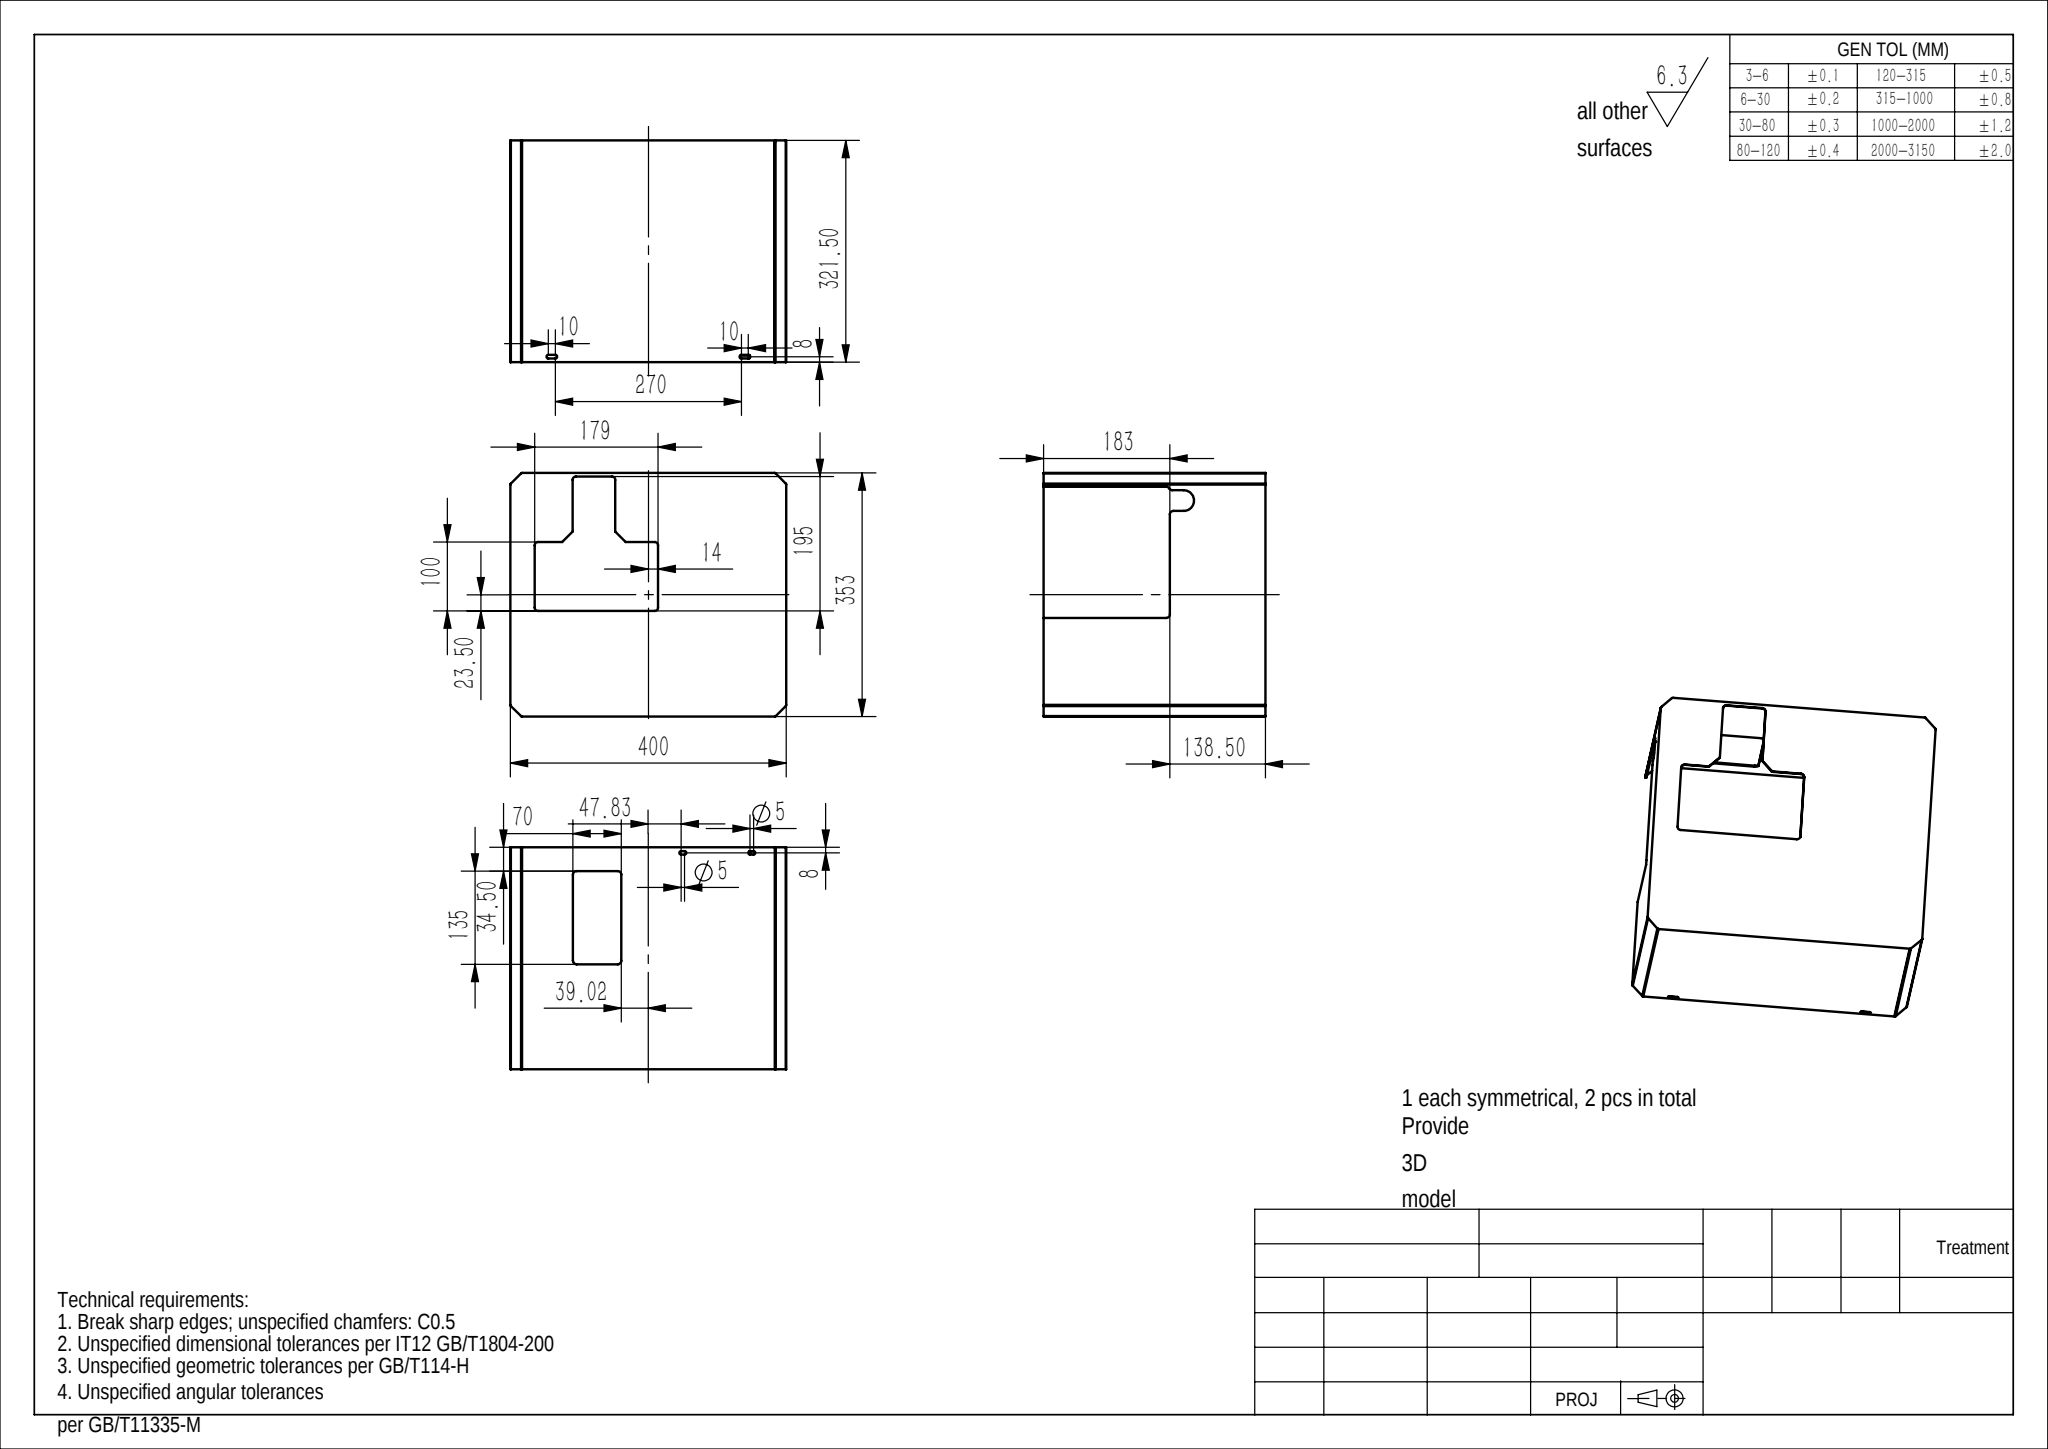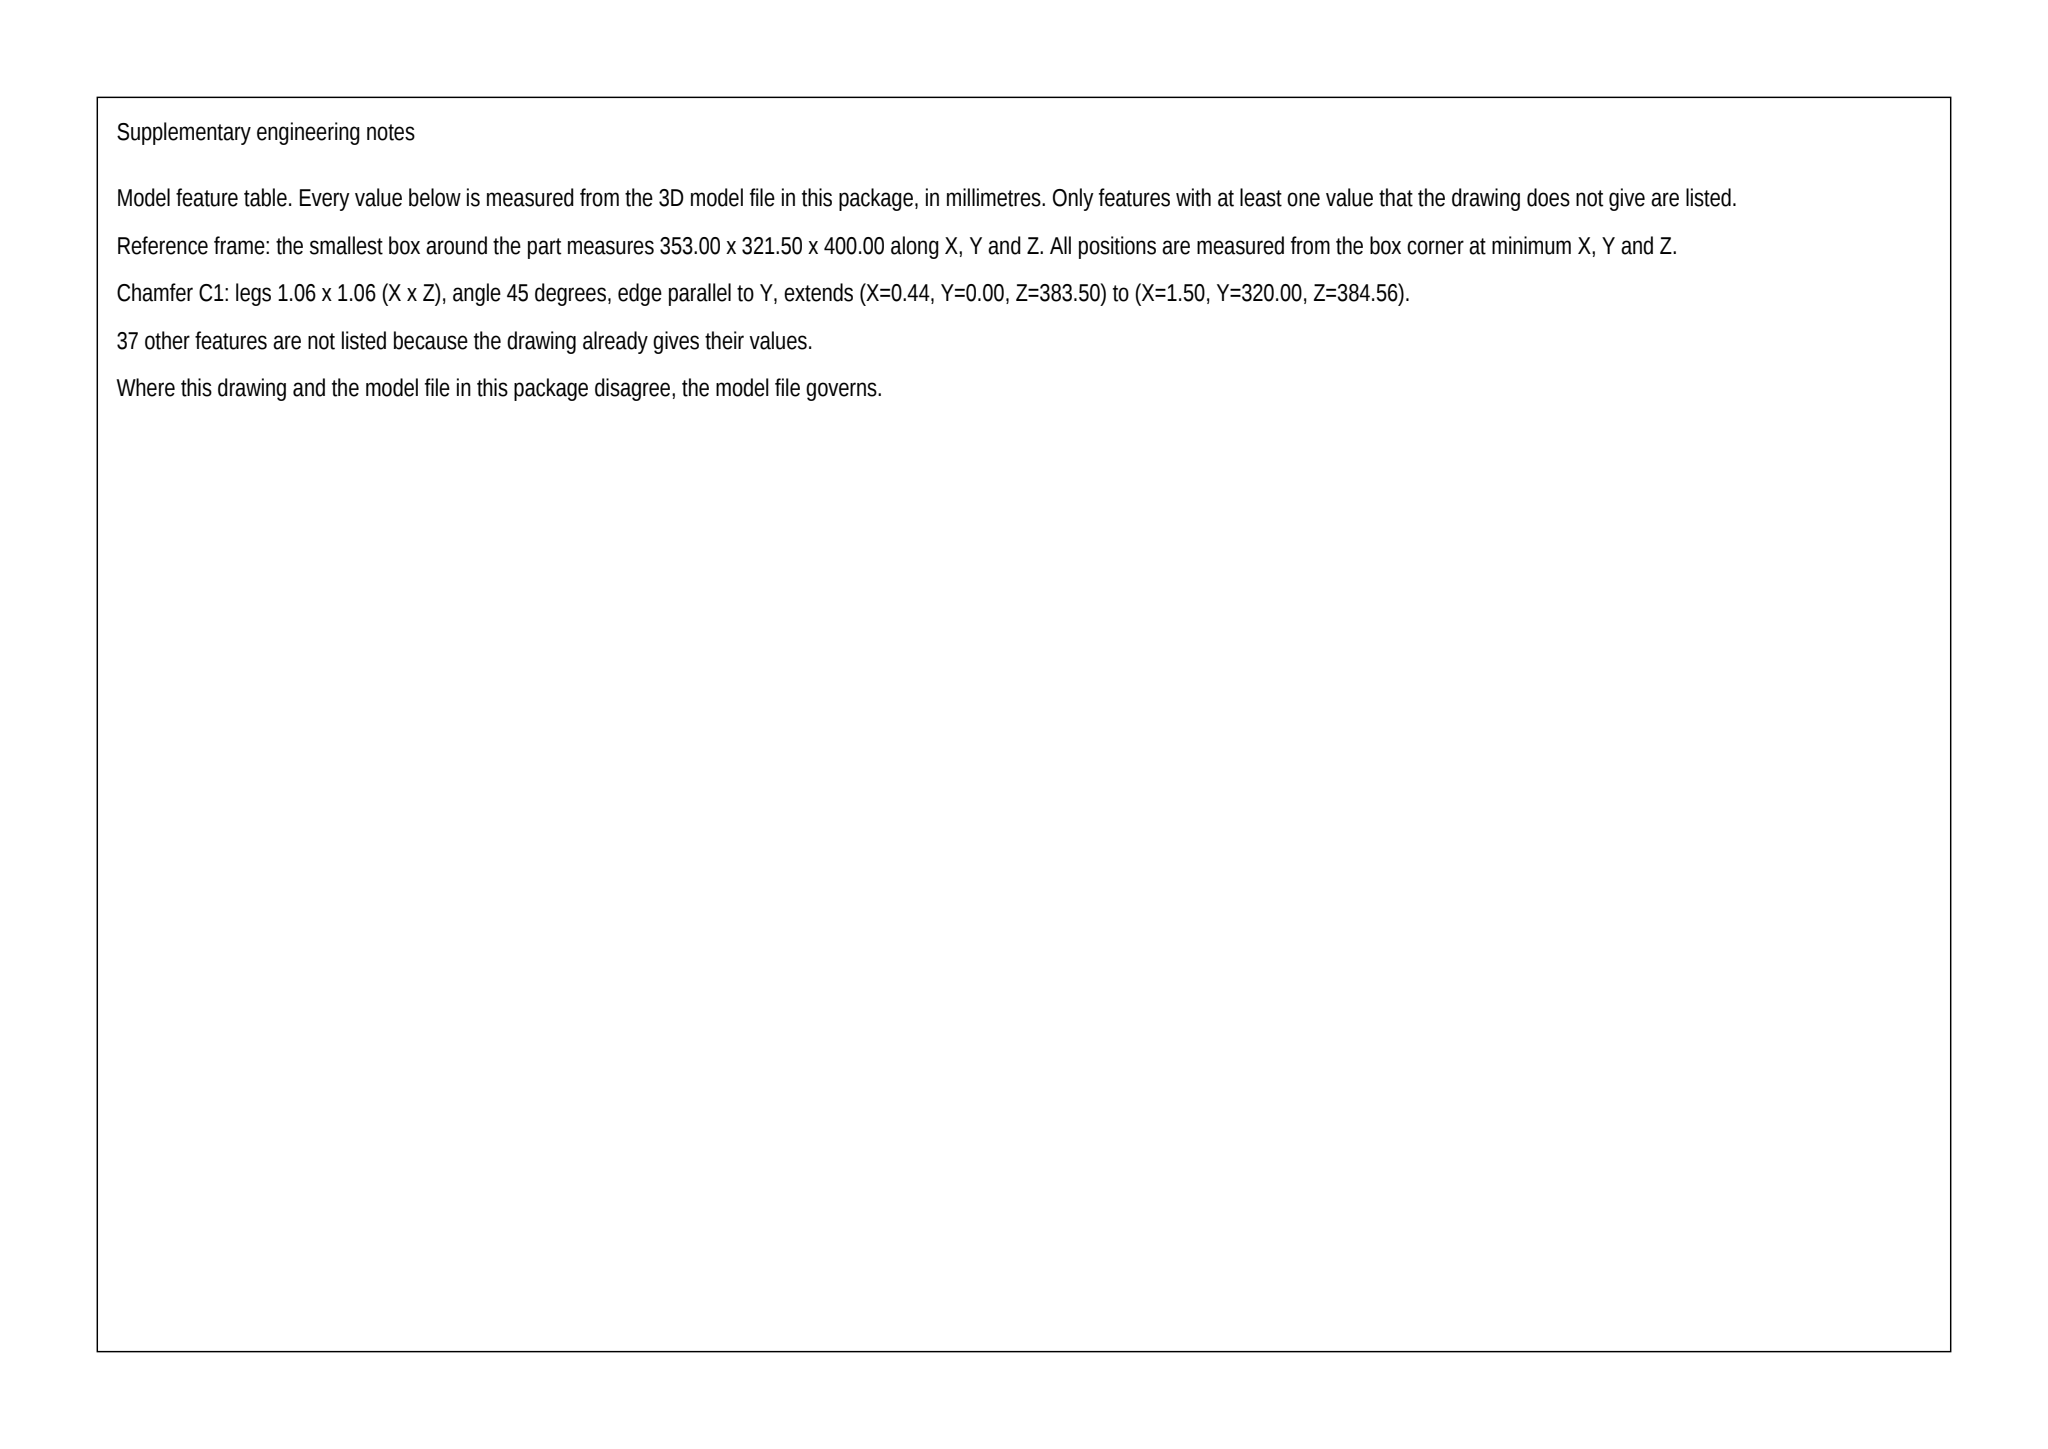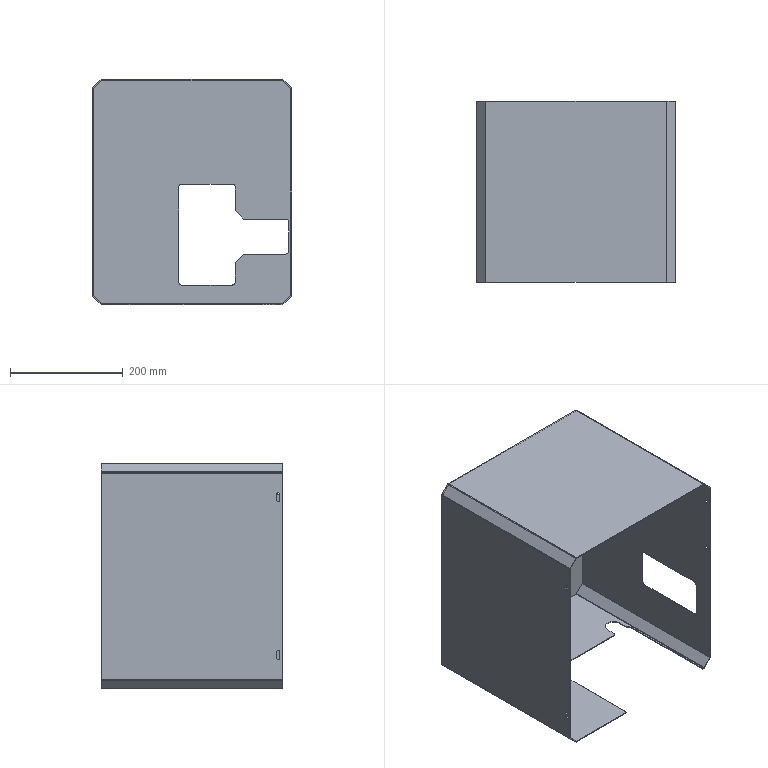Part | SolidWorks | mm | 1 solid | 104 faces | box 353 x 321.5 x 400 mm | volume 808617 mm3 | plane 63 | cylinder 41 | commonest cylinder face diameters 10 x14 1.473 x7 4.473 x7 5.5 x6 5 x6 30 x1